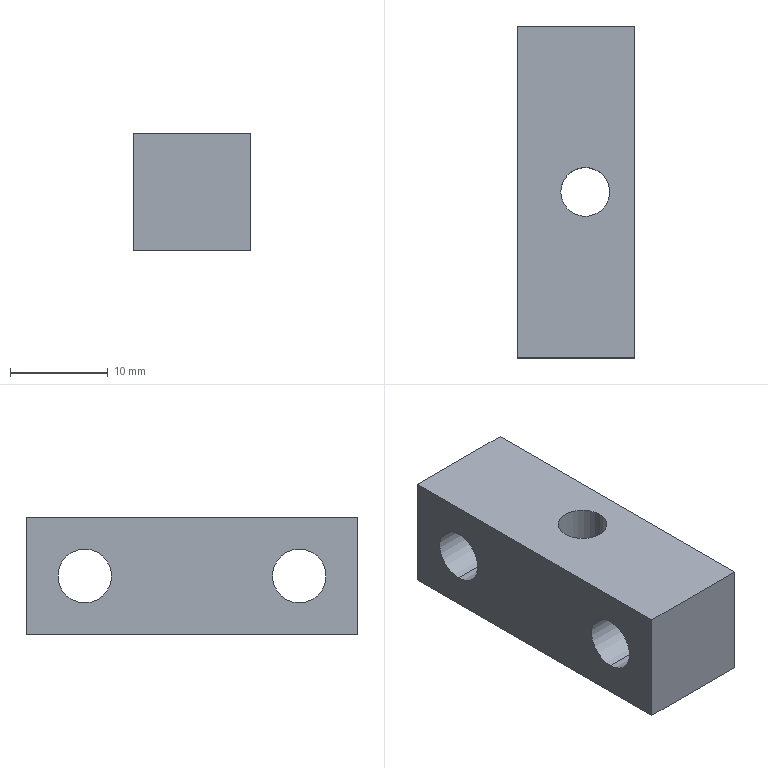Component | SolidWorks | CHEN123-AA-37-2 | 1 solid | 18 faces | box 12 x 34 x 12 mm | volume 3499 mm3 | cylinder 10 | plane 8 | commonest cylinder face diameters 10 x4 5.5 x4 5 x2
build123d program:
from build123d import *

# Parameters (mm, degrees)
SKETCH1_W                                       = 12
SKETCH1_H                                       = 34
BOSS_EXTRUDE1_DEPTH                             = 12
M6_TAPPED_HOLE1_D                               = 5
M5_HEX_SOCKET_HEAD_CAP_SCREW_CBORE1_D           = 5.5
M5_HEX_SOCKET_HEAD_CAP_SCREW_CBORE1_CBORE_D     = 10
M5_HEX_SOCKET_HEAD_CAP_SCREW_CBORE1_CBORE_DEPTH = 5.4


with BuildPart() as part:
    # Sketch1 → Boss-Extrude1 (new body)
    with BuildSketch(Plane.XY):
        Rectangle(SKETCH1_W, SKETCH1_H)
    extrude(amount=BOSS_EXTRUDE1_DEPTH)

    # M6 Tapped Hole1 (through all)
    with Locations(Plane(origin=(6, 0, 0), x_dir=(0, 0, -1), z_dir=(1, 0, 0))):
        with Locations((-6.948, 0)):
            Hole(M6_TAPPED_HOLE1_D / 2)

    # M5 Hex Socket Head Cap Screw CBORE1 (through all)
    with Locations(Plane.XY.offset(12)):
        with Locations((0, -11), (0, 11)):
            CounterBoreHole(M5_HEX_SOCKET_HEAD_CAP_SCREW_CBORE1_D / 2, M5_HEX_SOCKET_HEAD_CAP_SCREW_CBORE1_CBORE_D / 2, M5_HEX_SOCKET_HEAD_CAP_SCREW_CBORE1_CBORE_DEPTH)


solid = part.part

# Placed as in the assembly
solid = solid.moved(Location((28, -45.999, -156), (0, 90, 0)))
STEP:
#1=COLOUR_RGB('',0.7922,0.8196,0.9333);
#2=FILL_AREA_STYLE_COLOUR('',#1);
#3=FILL_AREA_STYLE('',(#2));
#4=SURFACE_STYLE_FILL_AREA(#3);
#5=SURFACE_SIDE_STYLE('',(#4));
#6=SURFACE_STYLE_USAGE(.BOTH.,#5);
#7=PRESENTATION_STYLE_ASSIGNMENT((#6));
#8=CARTESIAN_POINT('',(1.362,-2.244,-5.945));
#9=VERTEX_POINT('',#8);
#10=CARTESIAN_POINT('',(1.362,-2.244,-6.339));
#11=VERTEX_POINT('',#10);
#12=CARTESIAN_POINT('',(1.362,-2.244,-6.142));
#13=DIRECTION('',(1.,0.,0.));
#14=DIRECTION('',(0.,0.,-1.));
#15=AXIS2_PLACEMENT_3D('',#12,#13,#14);
#16=CIRCLE('',#15,0.1969);
#17=EDGE_CURVE('',#9,#11,#16,.T.);
#18=ORIENTED_EDGE('',*,*,#17,.F.);
#19=CARTESIAN_POINT('',(1.575,-2.244,-5.945));
#20=VERTEX_POINT('',#19);
#21=CARTESIAN_POINT('',(1.575,-2.244,-5.945));
#22=DIRECTION('',(1.,0.,0.));
#23=VECTOR('',#22,39.37);
#24=LINE('',#21,#23);
#25=EDGE_CURVE('',#9,#20,#24,.T.);
#26=ORIENTED_EDGE('',*,*,#25,.T.);
#27=CARTESIAN_POINT('',(1.575,-2.244,-6.339));
#28=VERTEX_POINT('',#27);
#29=CARTESIAN_POINT('',(1.575,-2.244,-6.142));
#30=DIRECTION('',(1.,0.,0.));
#31=DIRECTION('',(0.,0.,-1.));
#32=AXIS2_PLACEMENT_3D('',#29,#30,#31);
#33=CIRCLE('',#32,0.1969);
#34=EDGE_CURVE('',#20,#28,#33,.T.);
#35=ORIENTED_EDGE('',*,*,#34,.T.);
#36=CARTESIAN_POINT('',(1.575,-2.244,-6.339));
#37=DIRECTION('',(1.,0.,0.));
#38=VECTOR('',#37,39.37);
#39=LINE('',#36,#38);
#40=EDGE_CURVE('',#11,#28,#39,.T.);
#41=ORIENTED_EDGE('',*,*,#40,.F.);
#42=EDGE_LOOP('',(#18,#26,#35,#41));
#43=FACE_OUTER_BOUND('',#42,.T.);
#44=CARTESIAN_POINT('',(1.575,-2.244,-6.142));
#45=DIRECTION('',(1.,0.,0.));
#46=DIRECTION('',(0.,0.,-1.));
#47=AXIS2_PLACEMENT_3D('',#44,#45,#46);
#48=CYLINDRICAL_SURFACE('',#47,0.1969);
#49=ADVANCED_FACE('',(#43),#48,.F.);
#50=CARTESIAN_POINT('',(1.102,-2.244,-6.033));
#51=VERTEX_POINT('',#50);
#52=CARTESIAN_POINT('',(1.102,-2.244,-6.25));
#53=VERTEX_POINT('',#52);
#54=CARTESIAN_POINT('',(1.102,-2.244,-6.142));
#55=DIRECTION('',(1.,0.,0.));
#56=DIRECTION('',(0.,0.,-1.));
#57=AXIS2_PLACEMENT_3D('',#54,#55,#56);
#58=CIRCLE('',#57,0.1083);
#59=EDGE_CURVE('',#51,#53,#58,.T.);
#60=ORIENTED_EDGE('',*,*,#59,.F.);
#61=CARTESIAN_POINT('',(1.362,-2.244,-6.033));
#62=VERTEX_POINT('',#61);
#63=CARTESIAN_POINT('',(1.575,-2.244,-6.033));
#64=DIRECTION('',(1.,0.,0.));
#65=VECTOR('',#64,39.37);
#66=LINE('',#63,#65);
#67=EDGE_CURVE('',#51,#62,#66,.T.);
#68=ORIENTED_EDGE('',*,*,#67,.T.);
#69=CARTESIAN_POINT('',(1.362,-2.244,-6.25));
#70=VERTEX_POINT('',#69);
#71=CARTESIAN_POINT('',(1.362,-2.244,-6.142));
#72=DIRECTION('',(1.,0.,0.));
#73=DIRECTION('',(0.,0.,-1.));
#74=AXIS2_PLACEMENT_3D('',#71,#72,#73);
#75=CIRCLE('',#74,0.1083);
#76=EDGE_CURVE('',#62,#70,#75,.T.);
#77=ORIENTED_EDGE('',*,*,#76,.T.);
#78=CARTESIAN_POINT('',(1.575,-2.244,-6.25));
#79=DIRECTION('',(1.,0.,0.));
#80=VECTOR('',#79,39.37);
#81=LINE('',#78,#80);
#82=EDGE_CURVE('',#53,#70,#81,.T.);
#83=ORIENTED_EDGE('',*,*,#82,.F.);
#84=EDGE_LOOP('',(#60,#68,#77,#83));
#85=FACE_OUTER_BOUND('',#84,.T.);
#86=CARTESIAN_POINT('',(1.575,-2.244,-6.142));
#87=DIRECTION('',(1.,0.,0.));
#88=DIRECTION('',(0.,0.,-1.));
#89=AXIS2_PLACEMENT_3D('',#86,#87,#88);
#90=CYLINDRICAL_SURFACE('',#89,0.1083);
#91=ADVANCED_FACE('',(#85),#90,.F.);
#92=CARTESIAN_POINT('',(1.362,-1.378,-5.945));
#93=VERTEX_POINT('',#92);
#94=CARTESIAN_POINT('',(1.362,-1.378,-6.339));
#95=VERTEX_POINT('',#94);
#96=CARTESIAN_POINT('',(1.362,-1.378,-6.142));
#97=DIRECTION('',(1.,0.,0.));
#98=DIRECTION('',(0.,0.,-1.));
#99=AXIS2_PLACEMENT_3D('',#96,#97,#98);
#100=CIRCLE('',#99,0.1969);
#101=EDGE_CURVE('',#93,#95,#100,.T.);
#102=ORIENTED_EDGE('',*,*,#101,.F.);
#103=CARTESIAN_POINT('',(1.575,-1.378,-5.945));
#104=VERTEX_POINT('',#103);
#105=CARTESIAN_POINT('',(1.575,-1.378,-5.945));
#106=DIRECTION('',(1.,0.,0.));
#107=VECTOR('',#106,39.37);
#108=LINE('',#105,#107);
#109=EDGE_CURVE('',#93,#104,#108,.T.);
#110=ORIENTED_EDGE('',*,*,#109,.T.);
#111=CARTESIAN_POINT('',(1.575,-1.378,-6.339));
#112=VERTEX_POINT('',#111);
#113=CARTESIAN_POINT('',(1.575,-1.378,-6.142));
#114=DIRECTION('',(1.,0.,0.));
#115=DIRECTION('',(0.,0.,-1.));
#116=AXIS2_PLACEMENT_3D('',#113,#114,#115);
#117=CIRCLE('',#116,0.1969);
#118=EDGE_CURVE('',#104,#112,#117,.T.);
#119=ORIENTED_EDGE('',*,*,#118,.T.);
#120=CARTESIAN_POINT('',(1.575,-1.378,-6.339));
#121=DIRECTION('',(1.,0.,0.));
#122=VECTOR('',#121,39.37);
#123=LINE('',#120,#122);
#124=EDGE_CURVE('',#95,#112,#123,.T.);
#125=ORIENTED_EDGE('',*,*,#124,.F.);
#126=EDGE_LOOP('',(#102,#110,#119,#125));
#127=FACE_OUTER_BOUND('',#126,.T.);
#128=CARTESIAN_POINT('',(1.575,-1.378,-6.142));
#129=DIRECTION('',(1.,0.,0.));
#130=DIRECTION('',(0.,0.,-1.));
#131=AXIS2_PLACEMENT_3D('',#128,#129,#130);
#132=CYLINDRICAL_SURFACE('',#131,0.1969);
#133=ADVANCED_FACE('',(#127),#132,.F.);
#134=CARTESIAN_POINT('',(1.102,-1.378,-6.033));
#135=VERTEX_POINT('',#134);
#136=CARTESIAN_POINT('',(1.102,-1.378,-6.25));
#137=VERTEX_POINT('',#136);
#138=CARTESIAN_POINT('',(1.102,-1.378,-6.142));
#139=DIRECTION('',(1.,0.,0.));
#140=DIRECTION('',(0.,0.,-1.));
#141=AXIS2_PLACEMENT_3D('',#138,#139,#140);
#142=CIRCLE('',#141,0.1083);
#143=EDGE_CURVE('',#135,#137,#142,.T.);
#144=ORIENTED_EDGE('',*,*,#143,.F.);
#145=CARTESIAN_POINT('',(1.362,-1.378,-6.033));
#146=VERTEX_POINT('',#145);
#147=CARTESIAN_POINT('',(1.575,-1.378,-6.033));
#148=DIRECTION('',(1.,0.,0.));
#149=VECTOR('',#148,39.37);
#150=LINE('',#147,#149);
#151=EDGE_CURVE('',#135,#146,#150,.T.);
#152=ORIENTED_EDGE('',*,*,#151,.T.);
#153=CARTESIAN_POINT('',(1.362,-1.378,-6.25));
#154=VERTEX_POINT('',#153);
#155=CARTESIAN_POINT('',(1.362,-1.378,-6.142));
#156=DIRECTION('',(1.,0.,0.));
#157=DIRECTION('',(0.,0.,-1.));
#158=AXIS2_PLACEMENT_3D('',#155,#156,#157);
#159=CIRCLE('',#158,0.1083);
#160=EDGE_CURVE('',#146,#154,#159,.T.);
#161=ORIENTED_EDGE('',*,*,#160,.T.);
#162=CARTESIAN_POINT('',(1.575,-1.378,-6.25));
#163=DIRECTION('',(1.,0.,0.));
#164=VECTOR('',#163,39.37);
#165=LINE('',#162,#164);
#166=EDGE_CURVE('',#137,#154,#165,.T.);
#167=ORIENTED_EDGE('',*,*,#166,.F.);
#168=EDGE_LOOP('',(#144,#152,#161,#167));
#169=FACE_OUTER_BOUND('',#168,.T.);
#170=CARTESIAN_POINT('',(1.575,-1.378,-6.142));
#171=DIRECTION('',(1.,0.,0.));
#172=DIRECTION('',(0.,0.,-1.));
#173=AXIS2_PLACEMENT_3D('',#170,#171,#172);
#174=CYLINDRICAL_SURFACE('',#173,0.1083);
#175=ADVANCED_FACE('',(#169),#174,.F.);
#176=CARTESIAN_POINT('',(1.474,-1.811,-5.906));
#177=VERTEX_POINT('',#176);
#178=CARTESIAN_POINT('',(1.277,-1.811,-5.906));
#179=VERTEX_POINT('',#178);
#180=CARTESIAN_POINT('',(1.376,-1.811,-5.906));
#181=DIRECTION('',(0.,0.,-1.));
#182=DIRECTION('',(-1.,0.,0.));
#183=AXIS2_PLACEMENT_3D('',#180,#181,#182);
#184=CIRCLE('',#183,0.09843);
#185=EDGE_CURVE('',#177,#179,#184,.T.);
#186=ORIENTED_EDGE('',*,*,#185,.F.);
#187=CARTESIAN_POINT('',(1.474,-1.811,-6.378));
#188=VERTEX_POINT('',#187);
#189=CARTESIAN_POINT('',(1.474,-1.811,-6.378));
#190=DIRECTION('',(0.,0.,-1.));
#191=VECTOR('',#190,39.37);
#192=LINE('',#189,#191);
#193=EDGE_CURVE('',#177,#188,#192,.T.);
#194=ORIENTED_EDGE('',*,*,#193,.T.);
#195=CARTESIAN_POINT('',(1.277,-1.811,-6.378));
#196=VERTEX_POINT('',#195);
#197=CARTESIAN_POINT('',(1.376,-1.811,-6.378));
#198=DIRECTION('',(0.,0.,-1.));
#199=DIRECTION('',(-1.,0.,0.));
#200=AXIS2_PLACEMENT_3D('',#197,#198,#199);
#201=CIRCLE('',#200,0.09843);
#202=EDGE_CURVE('',#188,#196,#201,.T.);
#203=ORIENTED_EDGE('',*,*,#202,.T.);
#204=CARTESIAN_POINT('',(1.277,-1.811,-6.378));
#205=DIRECTION('',(0.,0.,-1.));
#206=VECTOR('',#205,39.37);
#207=LINE('',#204,#206);
#208=EDGE_CURVE('',#179,#196,#207,.T.);
#209=ORIENTED_EDGE('',*,*,#208,.F.);
#210=EDGE_LOOP('',(#186,#194,#203,#209));
#211=FACE_OUTER_BOUND('',#210,.T.);
#212=CARTESIAN_POINT('',(1.376,-1.811,-6.378));
#213=DIRECTION('',(0.,0.,-1.));
#214=DIRECTION('',(-1.,0.,0.));
#215=AXIS2_PLACEMENT_3D('',#212,#213,#214);
#216=CYLINDRICAL_SURFACE('',#215,0.09843);
#217=ADVANCED_FACE('',(#211),#216,.F.);
#218=CARTESIAN_POINT('',(1.376,-1.811,-6.378));
#219=DIRECTION('',(0.,0.,-1.));
#220=DIRECTION('',(-1.,0.,0.));
#221=AXIS2_PLACEMENT_3D('',#218,#219,#220);
#222=CIRCLE('',#221,0.09843);
#223=EDGE_CURVE('',#196,#188,#222,.T.);
#224=ORIENTED_EDGE('',*,*,#223,.F.);
#225=ORIENTED_EDGE('',*,*,#202,.F.);
#226=EDGE_LOOP('',(#224,#225));
#227=FACE_BOUND('',#226,.T.);
#228=CARTESIAN_POINT('',(1.102,-2.48,-6.378));
#229=VERTEX_POINT('',#228);
#230=CARTESIAN_POINT('',(1.102,-1.142,-6.378));
#231=VERTEX_POINT('',#230);
#232=CARTESIAN_POINT('',(1.102,-2.48,-6.378));
#233=DIRECTION('',(0.,1.,0.));
#234=VECTOR('',#233,39.37);
#235=LINE('',#232,#234);
#236=EDGE_CURVE('',#229,#231,#235,.T.);
#237=ORIENTED_EDGE('',*,*,#236,.T.);
#238=CARTESIAN_POINT('',(1.575,-1.142,-6.378));
#239=VERTEX_POINT('',#238);
#240=CARTESIAN_POINT('',(1.575,-1.142,-6.378));
#241=DIRECTION('',(-1.,0.,0.));
#242=VECTOR('',#241,39.37);
#243=LINE('',#240,#242);
#244=EDGE_CURVE('',#239,#231,#243,.T.);
#245=ORIENTED_EDGE('',*,*,#244,.F.);
#246=CARTESIAN_POINT('',(1.575,-2.48,-6.378));
#247=VERTEX_POINT('',#246);
#248=CARTESIAN_POINT('',(1.575,-2.48,-6.378));
#249=DIRECTION('',(0.,1.,0.));
#250=VECTOR('',#249,39.37);
#251=LINE('',#248,#250);
#252=EDGE_CURVE('',#247,#239,#251,.T.);
#253=ORIENTED_EDGE('',*,*,#252,.F.);
#254=CARTESIAN_POINT('',(1.575,-2.48,-6.378));
#255=DIRECTION('',(-1.,0.,0.));
#256=VECTOR('',#255,39.37);
#257=LINE('',#254,#256);
#258=EDGE_CURVE('',#247,#229,#257,.T.);
#259=ORIENTED_EDGE('',*,*,#258,.T.);
#260=EDGE_LOOP('',(#237,#245,#253,#259));
#261=FACE_OUTER_BOUND('',#260,.T.);
#262=CARTESIAN_POINT('',(1.575,-2.48,-6.378));
#263=DIRECTION('',(0.,0.,1.));
#264=DIRECTION('',(1.,0.,0.));
#265=AXIS2_PLACEMENT_3D('',#262,#263,#264);
#266=PLANE('',#265);
#267=ADVANCED_FACE('',(#227,#261),#266,.F.);
#268=CARTESIAN_POINT('',(1.102,-1.142,-5.906));
#269=VERTEX_POINT('',#268);
#270=CARTESIAN_POINT('',(1.102,-1.142,-5.906));
#271=DIRECTION('',(0.,0.,1.));
#272=VECTOR('',#271,39.37);
#273=LINE('',#270,#272);
#274=EDGE_CURVE('',#231,#269,#273,.T.);
#275=ORIENTED_EDGE('',*,*,#274,.T.);
#276=CARTESIAN_POINT('',(1.575,-1.142,-5.906));
#277=VERTEX_POINT('',#276);
#278=CARTESIAN_POINT('',(1.575,-1.142,-5.906));
#279=DIRECTION('',(-1.,0.,0.));
#280=VECTOR('',#279,39.37);
#281=LINE('',#278,#280);
#282=EDGE_CURVE('',#277,#269,#281,.T.);
#283=ORIENTED_EDGE('',*,*,#282,.F.);
#284=CARTESIAN_POINT('',(1.575,-1.142,-5.906));
#285=DIRECTION('',(0.,0.,1.));
#286=VECTOR('',#285,39.37);
#287=LINE('',#284,#286);
#288=EDGE_CURVE('',#239,#277,#287,.T.);
#289=ORIENTED_EDGE('',*,*,#288,.F.);
#290=ORIENTED_EDGE('',*,*,#244,.T.);
#291=EDGE_LOOP('',(#275,#283,#289,#290));
#292=FACE_OUTER_BOUND('',#291,.T.);
#293=CARTESIAN_POINT('',(1.575,-1.142,-5.906));
#294=DIRECTION('',(0.,-1.,0.));
#295=DIRECTION('',(-1.,0.,0.));
#296=AXIS2_PLACEMENT_3D('',#293,#294,#295);
#297=PLANE('',#296);
#298=ADVANCED_FACE('',(#292),#297,.F.);
#299=CARTESIAN_POINT('',(1.376,-1.811,-5.906));
#300=DIRECTION('',(0.,0.,-1.));
#301=DIRECTION('',(-1.,0.,0.));
#302=AXIS2_PLACEMENT_3D('',#299,#300,#301);
#303=CIRCLE('',#302,0.09843);
#304=EDGE_CURVE('',#179,#177,#303,.T.);
#305=ORIENTED_EDGE('',*,*,#304,.T.);
#306=ORIENTED_EDGE('',*,*,#185,.T.);
#307=EDGE_LOOP('',(#305,#306));
#308=FACE_BOUND('',#307,.T.);
#309=CARTESIAN_POINT('',(1.102,-2.48,-5.906));
#310=VERTEX_POINT('',#309);
#311=CARTESIAN_POINT('',(1.102,-2.48,-5.906));
#312=DIRECTION('',(0.,-1.,0.));
#313=VECTOR('',#312,39.37);
#314=LINE('',#311,#313);
#315=EDGE_CURVE('',#269,#310,#314,.T.);
#316=ORIENTED_EDGE('',*,*,#315,.T.);
#317=CARTESIAN_POINT('',(1.575,-2.48,-5.906));
#318=VERTEX_POINT('',#317);
#319=CARTESIAN_POINT('',(1.575,-2.48,-5.906));
#320=DIRECTION('',(-1.,0.,0.));
#321=VECTOR('',#320,39.37);
#322=LINE('',#319,#321);
#323=EDGE_CURVE('',#318,#310,#322,.T.);
#324=ORIENTED_EDGE('',*,*,#323,.F.);
#325=CARTESIAN_POINT('',(1.575,-2.48,-5.906));
#326=DIRECTION('',(0.,-1.,0.));
#327=VECTOR('',#326,39.37);
#328=LINE('',#325,#327);
#329=EDGE_CURVE('',#277,#318,#328,.T.);
#330=ORIENTED_EDGE('',*,*,#329,.F.);
#331=ORIENTED_EDGE('',*,*,#282,.T.);
#332=EDGE_LOOP('',(#316,#324,#330,#331));
#333=FACE_OUTER_BOUND('',#332,.T.);
#334=CARTESIAN_POINT('',(1.575,-2.48,-5.906));
#335=DIRECTION('',(0.,0.,-1.));
#336=DIRECTION('',(-1.,0.,0.));
#337=AXIS2_PLACEMENT_3D('',#334,#335,#336);
#338=PLANE('',#337);
#339=ADVANCED_FACE('',(#308,#333),#338,.F.);
#340=CARTESIAN_POINT('',(1.102,-2.48,-5.906));
#341=DIRECTION('',(0.,0.,-1.));
#342=VECTOR('',#341,39.37);
#343=LINE('',#340,#342);
#344=EDGE_CURVE('',#310,#229,#343,.T.);
#345=ORIENTED_EDGE('',*,*,#344,.T.);
#346=ORIENTED_EDGE('',*,*,#258,.F.);
#347=CARTESIAN_POINT('',(1.575,-2.48,-5.906));
#348=DIRECTION('',(0.,0.,-1.));
#349=VECTOR('',#348,39.37);
#350=LINE('',#347,#349);
#351=EDGE_CURVE('',#318,#247,#350,.T.);
#352=ORIENTED_EDGE('',*,*,#351,.F.);
#353=ORIENTED_EDGE('',*,*,#323,.T.);
#354=EDGE_LOOP('',(#345,#346,#352,#353));
#355=FACE_OUTER_BOUND('',#354,.T.);
#356=CARTESIAN_POINT('',(1.575,-2.48,-5.906));
#357=DIRECTION('',(0.,1.,0.));
#358=DIRECTION('',(1.,0.,0.));
#359=AXIS2_PLACEMENT_3D('',#356,#357,#358);
#360=PLANE('',#359);
#361=ADVANCED_FACE('',(#355),#360,.F.);
#362=CARTESIAN_POINT('',(1.575,-2.244,-6.142));
#363=DIRECTION('',(1.,0.,0.));
#364=DIRECTION('',(0.,0.,-1.));
#365=AXIS2_PLACEMENT_3D('',#362,#363,#364);
#366=CIRCLE('',#365,0.1969);
#367=EDGE_CURVE('',#28,#20,#366,.T.);
#368=ORIENTED_EDGE('',*,*,#367,.F.);
#369=ORIENTED_EDGE('',*,*,#34,.F.);
#370=EDGE_LOOP('',(#368,#369));
#371=FACE_BOUND('',#370,.T.);
#372=CARTESIAN_POINT('',(1.575,-1.378,-6.142));
#373=DIRECTION('',(1.,0.,0.));
#374=DIRECTION('',(0.,0.,-1.));
#375=AXIS2_PLACEMENT_3D('',#372,#373,#374);
#376=CIRCLE('',#375,0.1969);
#377=EDGE_CURVE('',#112,#104,#376,.T.);
#378=ORIENTED_EDGE('',*,*,#377,.F.);
#379=ORIENTED_EDGE('',*,*,#118,.F.);
#380=EDGE_LOOP('',(#378,#379));
#381=FACE_BOUND('',#380,.T.);
#382=ORIENTED_EDGE('',*,*,#252,.T.);
#383=ORIENTED_EDGE('',*,*,#288,.T.);
#384=ORIENTED_EDGE('',*,*,#329,.T.);
#385=ORIENTED_EDGE('',*,*,#351,.T.);
#386=EDGE_LOOP('',(#382,#383,#384,#385));
#387=FACE_OUTER_BOUND('',#386,.T.);
#388=CARTESIAN_POINT('',(1.575,-1.811,-6.142));
#389=DIRECTION('',(-1.,0.,0.));
#390=DIRECTION('',(0.,0.,1.));
#391=AXIS2_PLACEMENT_3D('',#388,#389,#390);
#392=PLANE('',#391);
#393=ADVANCED_FACE('',(#371,#381,#387),#392,.F.);
#394=CARTESIAN_POINT('',(1.102,-2.244,-6.142));
#395=DIRECTION('',(1.,0.,0.));
#396=DIRECTION('',(0.,0.,-1.));
#397=AXIS2_PLACEMENT_3D('',#394,#395,#396);
#398=CIRCLE('',#397,0.1083);
#399=EDGE_CURVE('',#53,#51,#398,.T.);
#400=ORIENTED_EDGE('',*,*,#399,.T.);
#401=ORIENTED_EDGE('',*,*,#59,.T.);
#402=EDGE_LOOP('',(#400,#401));
#403=FACE_BOUND('',#402,.T.);
#404=CARTESIAN_POINT('',(1.102,-1.378,-6.142));
#405=DIRECTION('',(1.,0.,0.));
#406=DIRECTION('',(0.,0.,-1.));
#407=AXIS2_PLACEMENT_3D('',#404,#405,#406);
#408=CIRCLE('',#407,0.1083);
#409=EDGE_CURVE('',#137,#135,#408,.T.);
#410=ORIENTED_EDGE('',*,*,#409,.T.);
#411=ORIENTED_EDGE('',*,*,#143,.T.);
#412=EDGE_LOOP('',(#410,#411));
#413=FACE_BOUND('',#412,.T.);
#414=ORIENTED_EDGE('',*,*,#236,.F.);
#415=ORIENTED_EDGE('',*,*,#344,.F.);
#416=ORIENTED_EDGE('',*,*,#315,.F.);
#417=ORIENTED_EDGE('',*,*,#274,.F.);
#418=EDGE_LOOP('',(#414,#415,#416,#417));
#419=FACE_OUTER_BOUND('',#418,.T.);
#420=CARTESIAN_POINT('',(1.102,-1.811,-6.142));
#421=DIRECTION('',(-1.,0.,0.));
#422=DIRECTION('',(0.,0.,1.));
#423=AXIS2_PLACEMENT_3D('',#420,#421,#422);
#424=PLANE('',#423);
#425=ADVANCED_FACE('',(#403,#413,#419),#424,.T.);
#426=ORIENTED_EDGE('',*,*,#193,.F.);
#427=ORIENTED_EDGE('',*,*,#304,.F.);
#428=ORIENTED_EDGE('',*,*,#208,.T.);
#429=ORIENTED_EDGE('',*,*,#223,.T.);
#430=EDGE_LOOP('',(#426,#427,#428,#429));
#431=FACE_OUTER_BOUND('',#430,.T.);
#432=CARTESIAN_POINT('',(1.376,-1.811,-6.378));
#433=DIRECTION('',(0.,0.,-1.));
#434=DIRECTION('',(-1.,0.,0.));
#435=AXIS2_PLACEMENT_3D('',#432,#433,#434);
#436=CYLINDRICAL_SURFACE('',#435,0.09843);
#437=ADVANCED_FACE('',(#431),#436,.F.);
#438=ORIENTED_EDGE('',*,*,#151,.F.);
#439=ORIENTED_EDGE('',*,*,#409,.F.);
#440=ORIENTED_EDGE('',*,*,#166,.T.);
#441=CARTESIAN_POINT('',(1.362,-1.378,-6.142));
#442=DIRECTION('',(1.,0.,0.));
#443=DIRECTION('',(0.,0.,-1.));
#444=AXIS2_PLACEMENT_3D('',#441,#442,#443);
#445=CIRCLE('',#444,0.1083);
#446=EDGE_CURVE('',#154,#146,#445,.T.);
#447=ORIENTED_EDGE('',*,*,#446,.T.);
#448=EDGE_LOOP('',(#438,#439,#440,#447));
#449=FACE_OUTER_BOUND('',#448,.T.);
#450=CARTESIAN_POINT('',(1.575,-1.378,-6.142));
#451=DIRECTION('',(1.,0.,0.));
#452=DIRECTION('',(0.,0.,-1.));
#453=AXIS2_PLACEMENT_3D('',#450,#451,#452);
#454=CYLINDRICAL_SURFACE('',#453,0.1083);
#455=ADVANCED_FACE('',(#449),#454,.F.);
#456=ORIENTED_EDGE('',*,*,#446,.F.);
#457=ORIENTED_EDGE('',*,*,#160,.F.);
#458=EDGE_LOOP('',(#456,#457));
#459=FACE_BOUND('',#458,.T.);
#460=CARTESIAN_POINT('',(1.362,-1.378,-6.142));
#461=DIRECTION('',(1.,0.,0.));
#462=DIRECTION('',(0.,0.,-1.));
#463=AXIS2_PLACEMENT_3D('',#460,#461,#462);
#464=CIRCLE('',#463,0.1969);
#465=EDGE_CURVE('',#95,#93,#464,.T.);
#466=ORIENTED_EDGE('',*,*,#465,.T.);
#467=ORIENTED_EDGE('',*,*,#101,.T.);
#468=EDGE_LOOP('',(#466,#467));
#469=FACE_OUTER_BOUND('',#468,.T.);
#470=CARTESIAN_POINT('',(1.362,-1.378,-6.25));
#471=DIRECTION('',(-1.,0.,0.));
#472=DIRECTION('',(0.,0.,1.));
#473=AXIS2_PLACEMENT_3D('',#470,#471,#472);
#474=PLANE('',#473);
#475=ADVANCED_FACE('',(#459,#469),#474,.F.);
#476=ORIENTED_EDGE('',*,*,#109,.F.);
#477=ORIENTED_EDGE('',*,*,#465,.F.);
#478=ORIENTED_EDGE('',*,*,#124,.T.);
#479=ORIENTED_EDGE('',*,*,#377,.T.);
#480=EDGE_LOOP('',(#476,#477,#478,#479));
#481=FACE_OUTER_BOUND('',#480,.T.);
#482=CARTESIAN_POINT('',(1.575,-1.378,-6.142));
#483=DIRECTION('',(1.,0.,0.));
#484=DIRECTION('',(0.,0.,-1.));
#485=AXIS2_PLACEMENT_3D('',#482,#483,#484);
#486=CYLINDRICAL_SURFACE('',#485,0.1969);
#487=ADVANCED_FACE('',(#481),#486,.F.);
#488=ORIENTED_EDGE('',*,*,#67,.F.);
#489=ORIENTED_EDGE('',*,*,#399,.F.);
#490=ORIENTED_EDGE('',*,*,#82,.T.);
#491=CARTESIAN_POINT('',(1.362,-2.244,-6.142));
#492=DIRECTION('',(1.,0.,0.));
#493=DIRECTION('',(0.,0.,-1.));
#494=AXIS2_PLACEMENT_3D('',#491,#492,#493);
#495=CIRCLE('',#494,0.1083);
#496=EDGE_CURVE('',#70,#62,#495,.T.);
#497=ORIENTED_EDGE('',*,*,#496,.T.);
#498=EDGE_LOOP('',(#488,#489,#490,#497));
#499=FACE_OUTER_BOUND('',#498,.T.);
#500=CARTESIAN_POINT('',(1.575,-2.244,-6.142));
#501=DIRECTION('',(1.,0.,0.));
#502=DIRECTION('',(0.,0.,-1.));
#503=AXIS2_PLACEMENT_3D('',#500,#501,#502);
#504=CYLINDRICAL_SURFACE('',#503,0.1083);
#505=ADVANCED_FACE('',(#499),#504,.F.);
#506=ORIENTED_EDGE('',*,*,#496,.F.);
#507=ORIENTED_EDGE('',*,*,#76,.F.);
#508=EDGE_LOOP('',(#506,#507));
#509=FACE_BOUND('',#508,.T.);
#510=CARTESIAN_POINT('',(1.362,-2.244,-6.142));
#511=DIRECTION('',(1.,0.,0.));
#512=DIRECTION('',(0.,0.,-1.));
#513=AXIS2_PLACEMENT_3D('',#510,#511,#512);
#514=CIRCLE('',#513,0.1969);
#515=EDGE_CURVE('',#11,#9,#514,.T.);
#516=ORIENTED_EDGE('',*,*,#515,.T.);
#517=ORIENTED_EDGE('',*,*,#17,.T.);
#518=EDGE_LOOP('',(#516,#517));
#519=FACE_OUTER_BOUND('',#518,.T.);
#520=CARTESIAN_POINT('',(1.362,-2.244,-6.25));
#521=DIRECTION('',(-1.,0.,0.));
#522=DIRECTION('',(0.,0.,1.));
#523=AXIS2_PLACEMENT_3D('',#520,#521,#522);
#524=PLANE('',#523);
#525=ADVANCED_FACE('',(#509,#519),#524,.F.);
#526=ORIENTED_EDGE('',*,*,#25,.F.);
#527=ORIENTED_EDGE('',*,*,#515,.F.);
#528=ORIENTED_EDGE('',*,*,#40,.T.);
#529=ORIENTED_EDGE('',*,*,#367,.T.);
#530=EDGE_LOOP('',(#526,#527,#528,#529));
#531=FACE_OUTER_BOUND('',#530,.T.);
#532=CARTESIAN_POINT('',(1.575,-2.244,-6.142));
#533=DIRECTION('',(1.,0.,0.));
#534=DIRECTION('',(0.,0.,-1.));
#535=AXIS2_PLACEMENT_3D('',#532,#533,#534);
#536=CYLINDRICAL_SURFACE('',#535,0.1969);
#537=ADVANCED_FACE('',(#531),#536,.F.);
#538=CLOSED_SHELL('',(#49,#91,#133,#175,#217,#267,#298,#339,#361,#393,#425,#437,#455,#475,#487,#505,#525,#537));
#539=MANIFOLD_SOLID_BREP('',#538);
#540=STYLED_ITEM('',(#7),#539);
#541=(LENGTH_UNIT()NAMED_UNIT(*)SI_UNIT($,.METRE.));
#542=LENGTH_MEASURE_WITH_UNIT(LENGTH_MEASURE(0.0254),#541);
#543=DIMENSIONAL_EXPONENTS(1.,0.,0.,0.,0.,0.,0.);
#544=(CONVERSION_BASED_UNIT('',#542)LENGTH_UNIT()NAMED_UNIT(#543));
#545=UNCERTAINTY_MEASURE_WITH_UNIT(LENGTH_MEASURE(0.00001),#544,'','');
#546=(NAMED_UNIT(*)PLANE_ANGLE_UNIT()SI_UNIT($,.RADIAN.));
#547=(NAMED_UNIT(*)SI_UNIT($,.STERADIAN.)SOLID_ANGLE_UNIT());
#548=(GEOMETRIC_REPRESENTATION_CONTEXT(3)GLOBAL_UNCERTAINTY_ASSIGNED_CONTEXT((#545))GLOBAL_UNIT_ASSIGNED_CONTEXT((#544,#546,#547))REPRESENTATION_CONTEXT('',''));
#549=MECHANICAL_DESIGN_GEOMETRIC_PRESENTATION_REPRESENTATION('',(#540),#548);
#550=PRESENTATION_LAYER_ASSIGNMENT('','',(#540));
#551=CARTESIAN_POINT('',(0.,0.,0.));
#552=DIRECTION('',(0.,0.,1.));
#553=DIRECTION('',(1.,0.,0.));
#554=AXIS2_PLACEMENT_3D('',#551,#552,#553);
#555=(LENGTH_UNIT()NAMED_UNIT(*)SI_UNIT($,.METRE.));
#556=LENGTH_MEASURE_WITH_UNIT(LENGTH_MEASURE(0.0254),#555);
#557=DIMENSIONAL_EXPONENTS(1.,0.,0.,0.,0.,0.,0.);
#558=(CONVERSION_BASED_UNIT('',#556)LENGTH_UNIT()NAMED_UNIT(#557));
#559=UNCERTAINTY_MEASURE_WITH_UNIT(LENGTH_MEASURE(0.00001),#558,'','');
#560=(NAMED_UNIT(*)PLANE_ANGLE_UNIT()SI_UNIT($,.RADIAN.));
#561=(NAMED_UNIT(*)SI_UNIT($,.STERADIAN.)SOLID_ANGLE_UNIT());
#562=(GEOMETRIC_REPRESENTATION_CONTEXT(3)GLOBAL_UNCERTAINTY_ASSIGNED_CONTEXT((#559))GLOBAL_UNIT_ASSIGNED_CONTEXT((#558,#560,#561))REPRESENTATION_CONTEXT('',''));
#563=ADVANCED_BREP_SHAPE_REPRESENTATION('',(#539,#554),#562);